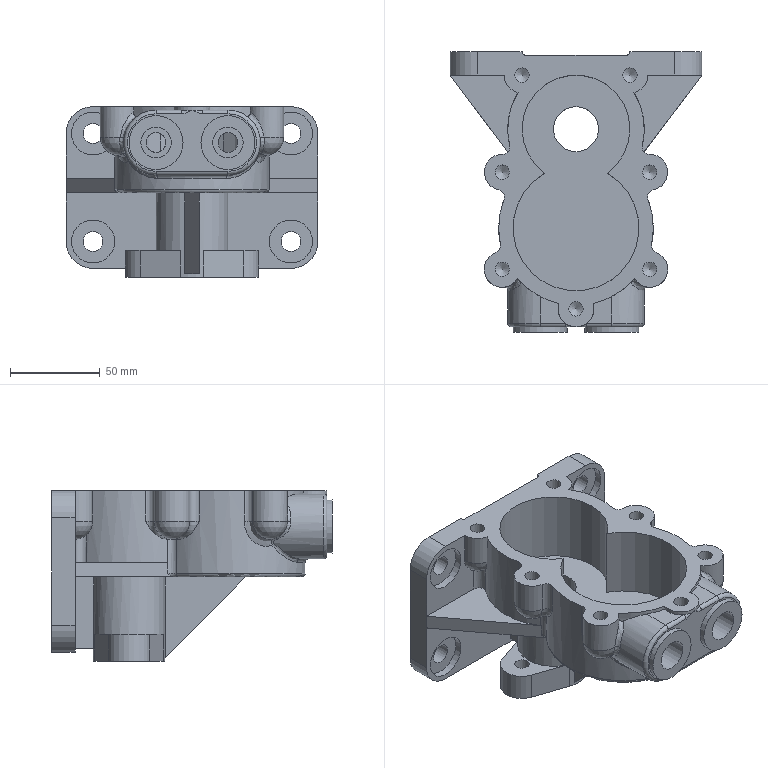Component | NX | 1_PUMP_BODY | 2 solids | 148 faces | volume 440826 mm3 | cylinder 65 | plane 48 | spline 12 | torus 10 | cone 7 | sphere 6 | commonest cylinder face diameters 8 x19 20 x9 30 x7 24 x6 11 x6 4 x5 86 x3 76 x2